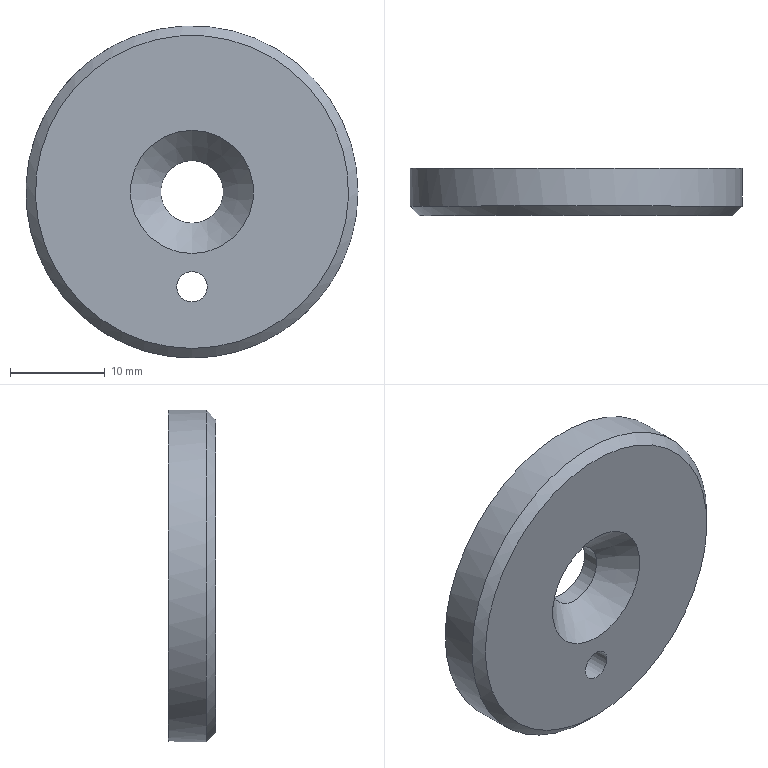Component | NX | CIRCLIP_35 | 1 solid | 7 faces | box 35 x 5 x 35 mm | volume 4405 mm3 | cylinder 3 | plane 2 | cone 2 | commonest cylinder face diameters 35 x1 6.6 x1 3.2 x1
STEP:
#1=CARTESIAN_POINT('',(0.,0.,0.));
#2=DIRECTION('',(0.,0.,1.));
#3=DIRECTION('',(1.,0.,0.));
#4=AXIS2_PLACEMENT_3D('',#1,#2,#3);
#5=CARTESIAN_POINT('',(378.803,-176.75,-152.5));
#6=VERTEX_POINT('',#5);
#7=CARTESIAN_POINT('',(396.303,-176.75,-135.));
#8=VERTEX_POINT('',#7);
#9=CARTESIAN_POINT('',(378.803,-176.75,-135.));
#10=DIRECTION('',(0.,1.,0.));
#11=DIRECTION('',(0.,0.,-1.));
#12=AXIS2_PLACEMENT_3D('',#9,#10,#11);
#13=CIRCLE('',#12,17.5);
#14=CARTESIAN_POINT('',(378.803,-177.75,-135.));
#15=DIRECTION('',(0.,1.,0.));
#16=DIRECTION('',(0.,0.,1.));
#17=AXIS2_PLACEMENT_3D('',#14,#15,#16);
#18=CYLINDRICAL_SURFACE('',#17,17.5);
#19=CARTESIAN_POINT('',(3.142,1.));
#20=DIRECTION('',(1.,0.));
#21=VECTOR('',#20,1.);
#22=LINE('',#19,#21);
#23=(GEOMETRIC_REPRESENTATION_CONTEXT(2)PARAMETRIC_REPRESENTATION_CONTEXT()REPRESENTATION_CONTEXT('',''));
#24=DEFINITIONAL_REPRESENTATION('',(#22),#23);
#25=PCURVE('',#18,#24);
#26=CARTESIAN_POINT('',(378.803,-177.75,-135.));
#27=DIRECTION('',(0.,1.,0.));
#28=DIRECTION('',(0.,0.,1.));
#29=AXIS2_PLACEMENT_3D('',#26,#27,#28);
#30=CONICAL_SURFACE('',#29,16.5,0.7854);
#31=CARTESIAN_POINT('',(3.142,1.));
#32=DIRECTION('',(1.,0.));
#33=VECTOR('',#32,1.);
#34=LINE('',#31,#33);
#35=(GEOMETRIC_REPRESENTATION_CONTEXT(2)PARAMETRIC_REPRESENTATION_CONTEXT()REPRESENTATION_CONTEXT('',''));
#36=DEFINITIONAL_REPRESENTATION('',(#34),#35);
#37=PCURVE('',#30,#36);
#38=SURFACE_CURVE('',#13,(#25,#37),.PCURVE_S1.);
#39=EDGE_CURVE('',#6,#8,#38,.T.);
#40=ORIENTED_EDGE('',*,*,#39,.T.);
#41=CARTESIAN_POINT('',(396.303,-172.75,-135.));
#42=VERTEX_POINT('',#41);
#43=CARTESIAN_POINT('',(396.303,-176.75,-135.));
#44=CARTESIAN_POINT('',(396.303,-172.75,-135.));
#45=B_SPLINE_CURVE_WITH_KNOTS('',1,(#43,#44),.UNSPECIFIED.,.F.,.F.,(2,2),(1.,5.),.PIECEWISE_BEZIER_KNOTS.);
#46=CARTESIAN_POINT('',(7.854,0.));
#47=DIRECTION('',(0.,1.));
#48=VECTOR('',#47,1.);
#49=LINE('',#46,#48);
#50=(GEOMETRIC_REPRESENTATION_CONTEXT(2)PARAMETRIC_REPRESENTATION_CONTEXT()REPRESENTATION_CONTEXT('',''));
#51=DEFINITIONAL_REPRESENTATION('',(#49),#50);
#52=PCURVE('',#18,#51);
#53=CARTESIAN_POINT('',(1.571,0.));
#54=DIRECTION('',(0.,1.));
#55=VECTOR('',#54,1.);
#56=LINE('',#53,#55);
#57=(GEOMETRIC_REPRESENTATION_CONTEXT(2)PARAMETRIC_REPRESENTATION_CONTEXT()REPRESENTATION_CONTEXT('',''));
#58=DEFINITIONAL_REPRESENTATION('',(#56),#57);
#59=PCURVE('',#18,#58);
#60=SEAM_CURVE('',#45,(#52,#59),.PCURVE_S1.);
#61=EDGE_CURVE('',#8,#42,#60,.T.);
#62=ORIENTED_EDGE('',*,*,#61,.T.);
#63=CARTESIAN_POINT('',(378.803,-172.75,-135.));
#64=DIRECTION('',(0.,-1.,0.));
#65=DIRECTION('',(1.,0.,0.));
#66=AXIS2_PLACEMENT_3D('',#63,#64,#65);
#67=CIRCLE('',#66,17.5);
#68=CARTESIAN_POINT('',(7.854,5.));
#69=DIRECTION('',(-1.,0.));
#70=VECTOR('',#69,1.);
#71=LINE('',#68,#70);
#72=(GEOMETRIC_REPRESENTATION_CONTEXT(2)PARAMETRIC_REPRESENTATION_CONTEXT()REPRESENTATION_CONTEXT('',''));
#73=DEFINITIONAL_REPRESENTATION('',(#71),#72);
#74=PCURVE('',#18,#73);
#75=CARTESIAN_POINT('',(378.803,-172.75,-135.));
#76=DIRECTION('',(0.,-1.,0.));
#77=DIRECTION('',(0.,0.,-1.));
#78=AXIS2_PLACEMENT_3D('',#75,#76,#77);
#79=PLANE('',#78);
#80=CARTESIAN_POINT('',(0.,0.));
#81=DIRECTION('',(0.,1.));
#82=AXIS2_PLACEMENT_2D('',#80,#81);
#83=CIRCLE('',#82,17.5);
#84=(GEOMETRIC_REPRESENTATION_CONTEXT(2)PARAMETRIC_REPRESENTATION_CONTEXT()REPRESENTATION_CONTEXT('',''));
#85=DEFINITIONAL_REPRESENTATION('',(#83),#84);
#86=PCURVE('',#79,#85);
#87=SURFACE_CURVE('',#67,(#74,#86),.PCURVE_S1.);
#88=EDGE_CURVE('',#42,#42,#87,.T.);
#89=ORIENTED_EDGE('',*,*,#88,.T.);
#90=ORIENTED_EDGE('',*,*,#61,.F.);
#91=CARTESIAN_POINT('',(378.803,-176.75,-135.));
#92=DIRECTION('',(0.,1.,0.));
#93=DIRECTION('',(0.,0.,-1.));
#94=AXIS2_PLACEMENT_3D('',#91,#92,#93);
#95=CIRCLE('',#94,17.5);
#96=CARTESIAN_POINT('',(-3.142,1.));
#97=DIRECTION('',(1.,0.));
#98=VECTOR('',#97,1.);
#99=LINE('',#96,#98);
#100=(GEOMETRIC_REPRESENTATION_CONTEXT(2)PARAMETRIC_REPRESENTATION_CONTEXT()REPRESENTATION_CONTEXT('',''));
#101=DEFINITIONAL_REPRESENTATION('',(#99),#100);
#102=PCURVE('',#18,#101);
#103=CARTESIAN_POINT('',(3.142,1.));
#104=DIRECTION('',(1.,0.));
#105=VECTOR('',#104,1.);
#106=LINE('',#103,#105);
#107=(GEOMETRIC_REPRESENTATION_CONTEXT(2)PARAMETRIC_REPRESENTATION_CONTEXT()REPRESENTATION_CONTEXT('',''));
#108=DEFINITIONAL_REPRESENTATION('',(#106),#107);
#109=PCURVE('',#30,#108);
#110=SURFACE_CURVE('',#95,(#102,#109),.PCURVE_S1.);
#111=EDGE_CURVE('',#8,#6,#110,.T.);
#112=ORIENTED_EDGE('',*,*,#111,.T.);
#113=EDGE_LOOP('',(#40,#62,#89,#90,#112));
#114=FACE_BOUND('',#113,.T.);
#115=ADVANCED_FACE('',(#114),#18,.T.);
#116=CARTESIAN_POINT('',(378.803,-177.75,-143.4));
#117=VERTEX_POINT('',#116);
#118=CARTESIAN_POINT('',(378.803,-177.75,-145.));
#119=DIRECTION('',(0.,1.,0.));
#120=DIRECTION('',(0.,0.,1.));
#121=AXIS2_PLACEMENT_3D('',#118,#119,#120);
#122=CIRCLE('',#121,1.6);
#123=CARTESIAN_POINT('',(378.803,-177.75,-135.));
#124=DIRECTION('',(0.,-1.,0.));
#125=DIRECTION('',(0.,0.,-1.));
#126=AXIS2_PLACEMENT_3D('',#123,#124,#125);
#127=PLANE('',#126);
#128=CARTESIAN_POINT('',(8.4,0.));
#129=CARTESIAN_POINT('',(8.4,2.771));
#130=CARTESIAN_POINT('',(10.8,1.386));
#131=CARTESIAN_POINT('',(13.2,0.));
#132=CARTESIAN_POINT('',(10.8,-1.386));
#133=CARTESIAN_POINT('',(8.4,-2.771));
#134=CARTESIAN_POINT('',(8.4,0.));
#135=(BOUNDED_CURVE()B_SPLINE_CURVE(2,(#128,#129,#130,#131,#132,#133,#134),.UNSPECIFIED.,.T.,.F.)B_SPLINE_CURVE_WITH_KNOTS((1,2,2,2,2,1),(-2.094,0.,2.094,4.189,6.283,8.378),.UNSPECIFIED.)CURVE()GEOMETRIC_REPRESENTATION_ITEM()RATIONAL_B_SPLINE_CURVE((1.,0.5,1.,0.5,1.,0.5,1.))REPRESENTATION_ITEM(''));
#136=(GEOMETRIC_REPRESENTATION_CONTEXT(2)PARAMETRIC_REPRESENTATION_CONTEXT()REPRESENTATION_CONTEXT('',''));
#137=DEFINITIONAL_REPRESENTATION('',(#135),#136);
#138=PCURVE('',#127,#137);
#139=CARTESIAN_POINT('',(378.803,-177.75,-145.));
#140=DIRECTION('',(0.,1.,0.));
#141=DIRECTION('',(0.,0.,1.));
#142=AXIS2_PLACEMENT_3D('',#139,#140,#141);
#143=CYLINDRICAL_SURFACE('',#142,1.6);
#144=CARTESIAN_POINT('',(0.,0.));
#145=DIRECTION('',(1.,0.));
#146=VECTOR('',#145,1.);
#147=LINE('',#144,#146);
#148=(GEOMETRIC_REPRESENTATION_CONTEXT(2)PARAMETRIC_REPRESENTATION_CONTEXT()REPRESENTATION_CONTEXT('',''));
#149=DEFINITIONAL_REPRESENTATION('',(#147),#148);
#150=PCURVE('',#143,#149);
#151=SURFACE_CURVE('',#122,(#138,#150),.PCURVE_S1.);
#152=EDGE_CURVE('',#117,#117,#151,.T.);
#153=ORIENTED_EDGE('',*,*,#152,.T.);
#154=EDGE_LOOP('',(#153));
#155=FACE_BOUND('',#154,.T.);
#156=CARTESIAN_POINT('',(378.803,-177.75,-151.5));
#157=VERTEX_POINT('',#156);
#158=CARTESIAN_POINT('',(378.803,-177.75,-135.));
#159=DIRECTION('',(0.,-1.,0.));
#160=DIRECTION('',(0.,0.,-1.));
#161=AXIS2_PLACEMENT_3D('',#158,#159,#160);
#162=CIRCLE('',#161,16.5);
#163=CARTESIAN_POINT('',(0.,0.));
#164=DIRECTION('',(1.,0.));
#165=AXIS2_PLACEMENT_2D('',#163,#164);
#166=CIRCLE('',#165,16.5);
#167=(GEOMETRIC_REPRESENTATION_CONTEXT(2)PARAMETRIC_REPRESENTATION_CONTEXT()REPRESENTATION_CONTEXT('',''));
#168=DEFINITIONAL_REPRESENTATION('',(#166),#167);
#169=PCURVE('',#127,#168);
#170=CARTESIAN_POINT('',(9.425,0.));
#171=DIRECTION('',(-1.,0.));
#172=VECTOR('',#171,1.);
#173=LINE('',#170,#172);
#174=(GEOMETRIC_REPRESENTATION_CONTEXT(2)PARAMETRIC_REPRESENTATION_CONTEXT()REPRESENTATION_CONTEXT('',''));
#175=DEFINITIONAL_REPRESENTATION('',(#173),#174);
#176=PCURVE('',#30,#175);
#177=SURFACE_CURVE('',#162,(#169,#176),.PCURVE_S1.);
#178=EDGE_CURVE('',#157,#157,#177,.T.);
#179=ORIENTED_EDGE('',*,*,#178,.T.);
#180=EDGE_LOOP('',(#179));
#181=FACE_BOUND('',#180,.T.);
#182=CARTESIAN_POINT('',(378.803,-177.75,-128.5));
#183=VERTEX_POINT('',#182);
#184=CARTESIAN_POINT('',(378.803,-177.75,-135.));
#185=DIRECTION('',(0.,1.,0.));
#186=DIRECTION('',(0.,0.,1.));
#187=AXIS2_PLACEMENT_3D('',#184,#185,#186);
#188=CIRCLE('',#187,6.5);
#189=CARTESIAN_POINT('',(-6.5,0.));
#190=CARTESIAN_POINT('',(-6.5,11.258));
#191=CARTESIAN_POINT('',(3.25,5.629));
#192=CARTESIAN_POINT('',(13.,0.));
#193=CARTESIAN_POINT('',(3.25,-5.629));
#194=CARTESIAN_POINT('',(-6.5,-11.258));
#195=CARTESIAN_POINT('',(-6.5,0.));
#196=(BOUNDED_CURVE()B_SPLINE_CURVE(2,(#189,#190,#191,#192,#193,#194,#195),.UNSPECIFIED.,.T.,.F.)B_SPLINE_CURVE_WITH_KNOTS((1,2,2,2,2,1),(-2.094,0.,2.094,4.189,6.283,8.378),.UNSPECIFIED.)CURVE()GEOMETRIC_REPRESENTATION_ITEM()RATIONAL_B_SPLINE_CURVE((1.,0.5,1.,0.5,1.,0.5,1.))REPRESENTATION_ITEM(''));
#197=(GEOMETRIC_REPRESENTATION_CONTEXT(2)PARAMETRIC_REPRESENTATION_CONTEXT()REPRESENTATION_CONTEXT('',''));
#198=DEFINITIONAL_REPRESENTATION('',(#196),#197);
#199=PCURVE('',#127,#198);
#200=CARTESIAN_POINT('',(378.803,-177.75,-135.));
#201=DIRECTION('',(0.,-1.,0.));
#202=DIRECTION('',(0.,0.,-1.));
#203=AXIS2_PLACEMENT_3D('',#200,#201,#202);
#204=CONICAL_SURFACE('',#203,6.5,0.7854);
#205=CARTESIAN_POINT('',(9.425,0.));
#206=DIRECTION('',(-1.,0.));
#207=VECTOR('',#206,1.);
#208=LINE('',#205,#207);
#209=(GEOMETRIC_REPRESENTATION_CONTEXT(2)PARAMETRIC_REPRESENTATION_CONTEXT()REPRESENTATION_CONTEXT('',''));
#210=DEFINITIONAL_REPRESENTATION('',(#208),#209);
#211=PCURVE('',#204,#210);
#212=SURFACE_CURVE('',#188,(#199,#211),.PCURVE_S1.);
#213=EDGE_CURVE('',#183,#183,#212,.T.);
#214=ORIENTED_EDGE('',*,*,#213,.T.);
#215=EDGE_LOOP('',(#214));
#216=FACE_BOUND('',#215,.T.);
#217=ADVANCED_FACE('',(#155,#181,#216),#127,.T.);
#218=CARTESIAN_POINT('',(378.803,-172.75,-146.6));
#219=VERTEX_POINT('',#218);
#220=CARTESIAN_POINT('',(378.803,-172.75,-143.4));
#221=VERTEX_POINT('',#220);
#222=CARTESIAN_POINT('',(378.803,-172.75,-145.));
#223=DIRECTION('',(0.,-1.,0.));
#224=DIRECTION('',(0.,0.,-1.));
#225=AXIS2_PLACEMENT_3D('',#222,#223,#224);
#226=CIRCLE('',#225,1.6);
#227=CARTESIAN_POINT('',(10.,0.));
#228=DIRECTION('',(1.,0.));
#229=AXIS2_PLACEMENT_2D('',#227,#228);
#230=CIRCLE('',#229,1.6);
#231=(GEOMETRIC_REPRESENTATION_CONTEXT(2)PARAMETRIC_REPRESENTATION_CONTEXT()REPRESENTATION_CONTEXT('',''));
#232=DEFINITIONAL_REPRESENTATION('',(#230),#231);
#233=PCURVE('',#79,#232);
#234=CARTESIAN_POINT('',(3.142,5.));
#235=DIRECTION('',(-1.,0.));
#236=VECTOR('',#235,1.);
#237=LINE('',#234,#236);
#238=(GEOMETRIC_REPRESENTATION_CONTEXT(2)PARAMETRIC_REPRESENTATION_CONTEXT()REPRESENTATION_CONTEXT('',''));
#239=DEFINITIONAL_REPRESENTATION('',(#237),#238);
#240=PCURVE('',#143,#239);
#241=SURFACE_CURVE('',#226,(#233,#240),.PCURVE_S1.);
#242=EDGE_CURVE('',#219,#221,#241,.T.);
#243=ORIENTED_EDGE('',*,*,#242,.T.);
#244=CARTESIAN_POINT('',(378.803,-172.75,-145.));
#245=DIRECTION('',(0.,-1.,0.));
#246=DIRECTION('',(0.,0.,-1.));
#247=AXIS2_PLACEMENT_3D('',#244,#245,#246);
#248=CIRCLE('',#247,1.6);
#249=CARTESIAN_POINT('',(10.,0.));
#250=DIRECTION('',(1.,0.));
#251=AXIS2_PLACEMENT_2D('',#249,#250);
#252=CIRCLE('',#251,1.6);
#253=(GEOMETRIC_REPRESENTATION_CONTEXT(2)PARAMETRIC_REPRESENTATION_CONTEXT()REPRESENTATION_CONTEXT('',''));
#254=DEFINITIONAL_REPRESENTATION('',(#252),#253);
#255=PCURVE('',#79,#254);
#256=CARTESIAN_POINT('',(9.425,5.));
#257=DIRECTION('',(-1.,0.));
#258=VECTOR('',#257,1.);
#259=LINE('',#256,#258);
#260=(GEOMETRIC_REPRESENTATION_CONTEXT(2)PARAMETRIC_REPRESENTATION_CONTEXT()REPRESENTATION_CONTEXT('',''));
#261=DEFINITIONAL_REPRESENTATION('',(#259),#260);
#262=PCURVE('',#143,#261);
#263=SURFACE_CURVE('',#248,(#255,#262),.PCURVE_S1.);
#264=EDGE_CURVE('',#221,#219,#263,.T.);
#265=ORIENTED_EDGE('',*,*,#264,.T.);
#266=EDGE_LOOP('',(#243,#265));
#267=FACE_BOUND('',#266,.T.);
#268=CARTESIAN_POINT('',(378.803,-172.75,-138.3));
#269=VERTEX_POINT('',#268);
#270=CARTESIAN_POINT('',(378.803,-172.75,-131.7));
#271=VERTEX_POINT('',#270);
#272=CARTESIAN_POINT('',(378.803,-172.75,-135.));
#273=DIRECTION('',(0.,-1.,0.));
#274=DIRECTION('',(0.,0.,-1.));
#275=AXIS2_PLACEMENT_3D('',#272,#273,#274);
#276=CIRCLE('',#275,3.3);
#277=CARTESIAN_POINT('',(0.,0.));
#278=DIRECTION('',(1.,0.));
#279=AXIS2_PLACEMENT_2D('',#277,#278);
#280=CIRCLE('',#279,3.3);
#281=(GEOMETRIC_REPRESENTATION_CONTEXT(2)PARAMETRIC_REPRESENTATION_CONTEXT()REPRESENTATION_CONTEXT('',''));
#282=DEFINITIONAL_REPRESENTATION('',(#280),#281);
#283=PCURVE('',#79,#282);
#284=CARTESIAN_POINT('',(378.803,494827.25,-135.));
#285=DIRECTION('',(0.,1.,0.));
#286=DIRECTION('',(0.,0.,1.));
#287=AXIS2_PLACEMENT_3D('',#284,#285,#286);
#288=CYLINDRICAL_SURFACE('',#287,3.3);
#289=CARTESIAN_POINT('',(3.142,-495000.));
#290=DIRECTION('',(-1.,0.));
#291=VECTOR('',#290,1.);
#292=LINE('',#289,#291);
#293=(GEOMETRIC_REPRESENTATION_CONTEXT(2)PARAMETRIC_REPRESENTATION_CONTEXT()REPRESENTATION_CONTEXT('',''));
#294=DEFINITIONAL_REPRESENTATION('',(#292),#293);
#295=PCURVE('',#288,#294);
#296=SURFACE_CURVE('',#276,(#283,#295),.PCURVE_S1.);
#297=EDGE_CURVE('',#269,#271,#296,.T.);
#298=ORIENTED_EDGE('',*,*,#297,.T.);
#299=CARTESIAN_POINT('',(378.803,-172.75,-135.));
#300=DIRECTION('',(0.,-1.,0.));
#301=DIRECTION('',(0.,0.,-1.));
#302=AXIS2_PLACEMENT_3D('',#299,#300,#301);
#303=CIRCLE('',#302,3.3);
#304=CARTESIAN_POINT('',(0.,0.));
#305=DIRECTION('',(1.,0.));
#306=AXIS2_PLACEMENT_2D('',#304,#305);
#307=CIRCLE('',#306,3.3);
#308=(GEOMETRIC_REPRESENTATION_CONTEXT(2)PARAMETRIC_REPRESENTATION_CONTEXT()REPRESENTATION_CONTEXT('',''));
#309=DEFINITIONAL_REPRESENTATION('',(#307),#308);
#310=PCURVE('',#79,#309);
#311=CARTESIAN_POINT('',(9.425,-495000.));
#312=DIRECTION('',(-1.,0.));
#313=VECTOR('',#312,1.);
#314=LINE('',#311,#313);
#315=(GEOMETRIC_REPRESENTATION_CONTEXT(2)PARAMETRIC_REPRESENTATION_CONTEXT()REPRESENTATION_CONTEXT('',''));
#316=DEFINITIONAL_REPRESENTATION('',(#314),#315);
#317=PCURVE('',#288,#316);
#318=SURFACE_CURVE('',#303,(#310,#317),.PCURVE_S1.);
#319=EDGE_CURVE('',#271,#269,#318,.T.);
#320=ORIENTED_EDGE('',*,*,#319,.T.);
#321=EDGE_LOOP('',(#298,#320));
#322=FACE_BOUND('',#321,.T.);
#323=ORIENTED_EDGE('',*,*,#88,.F.);
#324=EDGE_LOOP('',(#323));
#325=FACE_BOUND('',#324,.T.);
#326=ADVANCED_FACE('',(#267,#322,#325),#79,.F.);
#327=CARTESIAN_POINT('',(378.803,-174.55,-131.7));
#328=VERTEX_POINT('',#327);
#329=CARTESIAN_POINT('',(378.803,-174.55,-135.));
#330=DIRECTION('',(0.,-1.,0.));
#331=DIRECTION('',(0.,0.,1.));
#332=AXIS2_PLACEMENT_3D('',#329,#330,#331);
#333=CIRCLE('',#332,3.3);
#334=CARTESIAN_POINT('',(6.283,-495001.8));
#335=DIRECTION('',(-1.,0.));
#336=VECTOR('',#335,1.);
#337=LINE('',#334,#336);
#338=(GEOMETRIC_REPRESENTATION_CONTEXT(2)PARAMETRIC_REPRESENTATION_CONTEXT()REPRESENTATION_CONTEXT('',''));
#339=DEFINITIONAL_REPRESENTATION('',(#337),#338);
#340=PCURVE('',#288,#339);
#341=CARTESIAN_POINT('',(3.142,-3.2));
#342=DIRECTION('',(1.,0.));
#343=VECTOR('',#342,1.);
#344=LINE('',#341,#343);
#345=(GEOMETRIC_REPRESENTATION_CONTEXT(2)PARAMETRIC_REPRESENTATION_CONTEXT()REPRESENTATION_CONTEXT('',''));
#346=DEFINITIONAL_REPRESENTATION('',(#344),#345);
#347=PCURVE('',#204,#346);
#348=SURFACE_CURVE('',#333,(#340,#347),.PCURVE_S1.);
#349=EDGE_CURVE('',#328,#328,#348,.T.);
#350=ORIENTED_EDGE('',*,*,#349,.F.);
#351=CARTESIAN_POINT('',(378.803,-174.55,-131.7));
#352=CARTESIAN_POINT('',(378.803,-172.75,-131.7));
#353=B_SPLINE_CURVE_WITH_KNOTS('',1,(#351,#352),.UNSPECIFIED.,.F.,.F.,(2,2),(-495001.8,-495000.),.PIECEWISE_BEZIER_KNOTS.);
#354=CARTESIAN_POINT('',(6.283,0.));
#355=DIRECTION('',(0.,1.));
#356=VECTOR('',#355,1.);
#357=LINE('',#354,#356);
#358=(GEOMETRIC_REPRESENTATION_CONTEXT(2)PARAMETRIC_REPRESENTATION_CONTEXT()REPRESENTATION_CONTEXT('',''));
#359=DEFINITIONAL_REPRESENTATION('',(#357),#358);
#360=PCURVE('',#288,#359);
#361=CARTESIAN_POINT('',(0.,0.));
#362=DIRECTION('',(0.,1.));
#363=VECTOR('',#362,1.);
#364=LINE('',#361,#363);
#365=(GEOMETRIC_REPRESENTATION_CONTEXT(2)PARAMETRIC_REPRESENTATION_CONTEXT()REPRESENTATION_CONTEXT('',''));
#366=DEFINITIONAL_REPRESENTATION('',(#364),#365);
#367=PCURVE('',#288,#366);
#368=SEAM_CURVE('',#353,(#360,#367),.PCURVE_S1.);
#369=EDGE_CURVE('',#328,#271,#368,.T.);
#370=ORIENTED_EDGE('',*,*,#369,.T.);
#371=ORIENTED_EDGE('',*,*,#319,.T.);
#372=ORIENTED_EDGE('',*,*,#297,.T.);
#373=ORIENTED_EDGE('',*,*,#369,.F.);
#374=EDGE_LOOP('',(#350,#370,#371,#372,#373));
#375=FACE_BOUND('',#374,.F.);
#376=ADVANCED_FACE('',(#375),#288,.F.);
#377=ORIENTED_EDGE('',*,*,#349,.T.);
#378=CARTESIAN_POINT('',(378.803,-174.55,-131.7));
#379=CARTESIAN_POINT('',(378.803,-177.75,-128.5));
#380=B_SPLINE_CURVE_WITH_KNOTS('',1,(#378,#379),.UNSPECIFIED.,.F.,.F.,(2,2),(-4.525,0.),.PIECEWISE_BEZIER_KNOTS.);
#381=CARTESIAN_POINT('',(9.425,0.));
#382=DIRECTION('',(0.,1.));
#383=VECTOR('',#382,1.);
#384=LINE('',#381,#383);
#385=(GEOMETRIC_REPRESENTATION_CONTEXT(2)PARAMETRIC_REPRESENTATION_CONTEXT()REPRESENTATION_CONTEXT('',''));
#386=DEFINITIONAL_REPRESENTATION('',(#384),#385);
#387=PCURVE('',#204,#386);
#388=CARTESIAN_POINT('',(3.142,0.));
#389=DIRECTION('',(0.,1.));
#390=VECTOR('',#389,1.);
#391=LINE('',#388,#390);
#392=(GEOMETRIC_REPRESENTATION_CONTEXT(2)PARAMETRIC_REPRESENTATION_CONTEXT()REPRESENTATION_CONTEXT('',''));
#393=DEFINITIONAL_REPRESENTATION('',(#391),#392);
#394=PCURVE('',#204,#393);
#395=SEAM_CURVE('',#380,(#387,#394),.PCURVE_S1.);
#396=EDGE_CURVE('',#328,#183,#395,.T.);
#397=ORIENTED_EDGE('',*,*,#396,.T.);
#398=ORIENTED_EDGE('',*,*,#213,.T.);
#399=ORIENTED_EDGE('',*,*,#396,.F.);
#400=EDGE_LOOP('',(#377,#397,#398,#399));
#401=FACE_BOUND('',#400,.F.);
#402=ADVANCED_FACE('',(#401),#204,.F.);
#403=ORIENTED_EDGE('',*,*,#39,.F.);
#404=CARTESIAN_POINT('',(378.803,-177.75,-151.5));
#405=CARTESIAN_POINT('',(378.803,-176.75,-152.5));
#406=B_SPLINE_CURVE_WITH_KNOTS('',1,(#404,#405),.UNSPECIFIED.,.F.,.F.,(2,2),(0.,1.414),.PIECEWISE_BEZIER_KNOTS.);
#407=CARTESIAN_POINT('',(3.142,0.));
#408=DIRECTION('',(0.,1.));
#409=VECTOR('',#408,1.);
#410=LINE('',#407,#409);
#411=(GEOMETRIC_REPRESENTATION_CONTEXT(2)PARAMETRIC_REPRESENTATION_CONTEXT()REPRESENTATION_CONTEXT('',''));
#412=DEFINITIONAL_REPRESENTATION('',(#410),#411);
#413=PCURVE('',#30,#412);
#414=CARTESIAN_POINT('',(9.425,0.));
#415=DIRECTION('',(0.,1.));
#416=VECTOR('',#415,1.);
#417=LINE('',#414,#416);
#418=(GEOMETRIC_REPRESENTATION_CONTEXT(2)PARAMETRIC_REPRESENTATION_CONTEXT()REPRESENTATION_CONTEXT('',''));
#419=DEFINITIONAL_REPRESENTATION('',(#417),#418);
#420=PCURVE('',#30,#419);
#421=SEAM_CURVE('',#406,(#413,#420),.PCURVE_S1.);
#422=EDGE_CURVE('',#157,#6,#421,.T.);
#423=ORIENTED_EDGE('',*,*,#422,.F.);
#424=ORIENTED_EDGE('',*,*,#178,.F.);
#425=ORIENTED_EDGE('',*,*,#422,.T.);
#426=ORIENTED_EDGE('',*,*,#111,.F.);
#427=EDGE_LOOP('',(#403,#423,#424,#425,#426));
#428=FACE_BOUND('',#427,.T.);
#429=ADVANCED_FACE('',(#428),#30,.T.);
#430=ORIENTED_EDGE('',*,*,#152,.T.);
#431=CARTESIAN_POINT('',(378.803,-177.75,-143.4));
#432=CARTESIAN_POINT('',(378.803,-172.75,-143.4));
#433=B_SPLINE_CURVE_WITH_KNOTS('',1,(#431,#432),.UNSPECIFIED.,.F.,.F.,(2,2),(0.,5.),.PIECEWISE_BEZIER_KNOTS.);
#434=CARTESIAN_POINT('',(6.283,0.));
#435=DIRECTION('',(0.,1.));
#436=VECTOR('',#435,1.);
#437=LINE('',#434,#436);
#438=(GEOMETRIC_REPRESENTATION_CONTEXT(2)PARAMETRIC_REPRESENTATION_CONTEXT()REPRESENTATION_CONTEXT('',''));
#439=DEFINITIONAL_REPRESENTATION('',(#437),#438);
#440=PCURVE('',#143,#439);
#441=CARTESIAN_POINT('',(0.,0.));
#442=DIRECTION('',(0.,1.));
#443=VECTOR('',#442,1.);
#444=LINE('',#441,#443);
#445=(GEOMETRIC_REPRESENTATION_CONTEXT(2)PARAMETRIC_REPRESENTATION_CONTEXT()REPRESENTATION_CONTEXT('',''));
#446=DEFINITIONAL_REPRESENTATION('',(#444),#445);
#447=PCURVE('',#143,#446);
#448=SEAM_CURVE('',#433,(#440,#447),.PCURVE_S1.);
#449=EDGE_CURVE('',#117,#221,#448,.T.);
#450=ORIENTED_EDGE('',*,*,#449,.T.);
#451=ORIENTED_EDGE('',*,*,#264,.T.);
#452=ORIENTED_EDGE('',*,*,#242,.T.);
#453=ORIENTED_EDGE('',*,*,#449,.F.);
#454=EDGE_LOOP('',(#430,#450,#451,#452,#453));
#455=FACE_BOUND('',#454,.F.);
#456=ADVANCED_FACE('',(#455),#143,.F.);
#457=CLOSED_SHELL('',(#115,#217,#326,#376,#402,#429,#456));
#458=MANIFOLD_SOLID_BREP('',#457);
#459=(LENGTH_UNIT()NAMED_UNIT(*)SI_UNIT(.MILLI.,.METRE.));
#460=UNCERTAINTY_MEASURE_WITH_UNIT(LENGTH_MEASURE(0.000005),#459,'','');
#461=(NAMED_UNIT(*)PLANE_ANGLE_UNIT()SI_UNIT($,.RADIAN.));
#462=(NAMED_UNIT(*)SI_UNIT($,.STERADIAN.)SOLID_ANGLE_UNIT());
#463=(GEOMETRIC_REPRESENTATION_CONTEXT(3)GLOBAL_UNCERTAINTY_ASSIGNED_CONTEXT((#460))GLOBAL_UNIT_ASSIGNED_CONTEXT((#459,#461,#462))REPRESENTATION_CONTEXT('',''));
#464=ADVANCED_BREP_SHAPE_REPRESENTATION('',(#4,#458),#463);